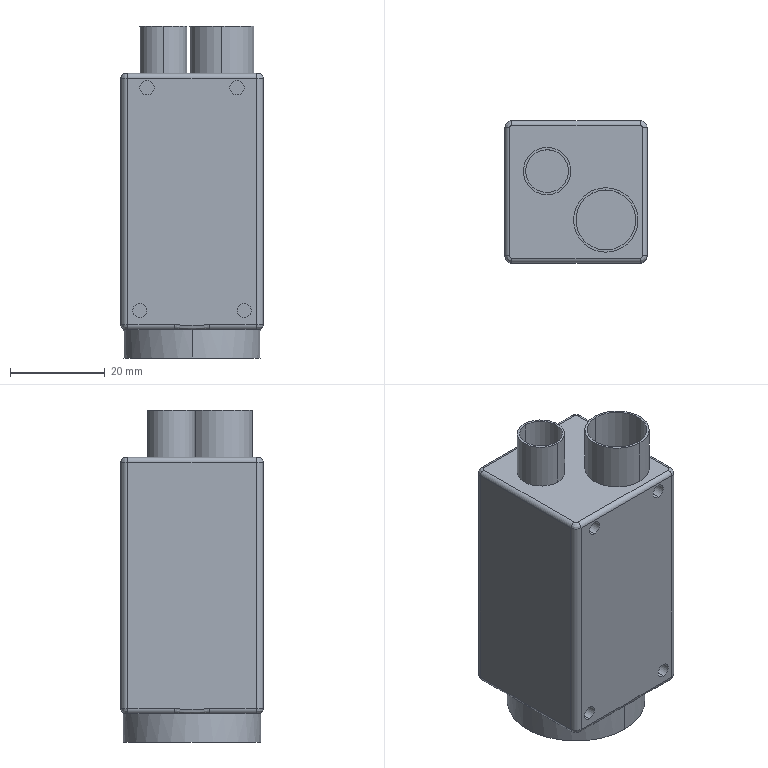Component | SolidWorks | connex1100-1 | 1 solid | 67 faces | volume 49431 mm3 | cylinder 36 | plane 19 | spline 12 | commonest cylinder face diameters 3 x12 2 x12 29 x2 10 x2 13.6 x2 26.211 x2 9.025 x2 12.641 x2